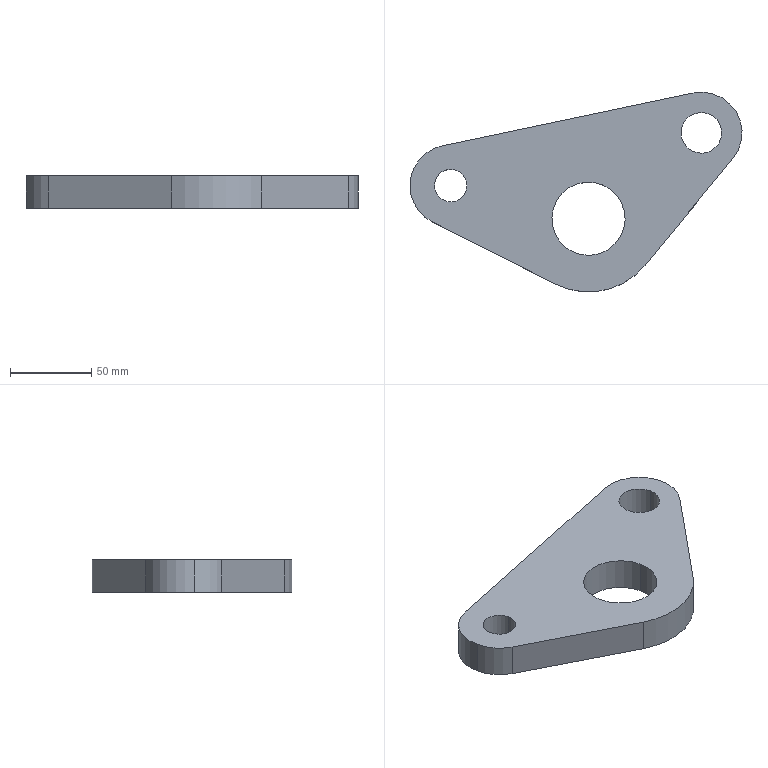Component | SolidWorks | TriangularCrank1-1 | 1 solid | 15 faces | box 204.08 x 122.79 x 20 mm | volume 266584 mm3 | cylinder 10 | plane 5 | commonest cylinder face diameters 50 x3 25 x2 20 x2 45 x2 90 x1 | material N/A
build123d program:
from build123d import *

# Parameters (mm, degrees)
BOSS_EXTRUDE1_DEPTH    = 10
FILLET1_R              = 45
SKETCH2_R              = 22.5
CUT_EXTRUDE1_DEPTH     = 186.55
FILLET2_R              = 25
M20_TAPPED_HOLE1_D     = 20
M20_TAPPED_HOLE1_DEPTH = 47.5
M20_TAPPED_HOLE1_TIP   = 6.009
SKETCH5_R              = 12.5
CUT_EXTRUDE2_DEPTH     = 151.628


with BuildPart() as part:
    # Sketch1 → Boss-Extrude1 (new, symmetric)
    with BuildSketch(Plane(origin=(0, 0, 0), x_dir=(0, 0, -1), z_dir=(1, 0, 0))):
        Polygon((-150, 0), (150, 0), (0, -120), align=None)
    extrude(amount=BOSS_EXTRUDE1_DEPTH, both=True)

    # Fillet1
    fillet1_edges = [part.edges().sort_by_distance(p)[0] for p in [
        (0, -120, 0),
    ]]
    fillet(fillet1_edges, radius=FILLET1_R)

    # Sketch2 → Cut-Extrude1 (cut, through all)
    with BuildSketch(Plane(origin=(10, 0, 0), x_dir=(0, 0, -1), z_dir=(1, 0, 0))):
        with Locations((0, -62.372)):
            Circle(SKETCH2_R)
    extrude(amount=-CUT_EXTRUDE1_DEPTH, mode=Mode.SUBTRACT)

    # Fillet2
    fillet2_edges = [part.edges().sort_by_distance(p)[0] for p in [
        (0, 0, 150),
        (0, 0, -150),
    ]]
    fillet(fillet2_edges, radius=FILLET2_R)

    # M20 Tapped Hole1
    with Locations(Plane(origin=(10, 0, 0), x_dir=(0, 0, -1), z_dir=(1, 0, 0))):
        with Locations((-78.73, -25), (78.73, -25)):
            Hole(M20_TAPPED_HOLE1_D / 2, depth=M20_TAPPED_HOLE1_DEPTH)
            with Locations((0, 0, -(M20_TAPPED_HOLE1_DEPTH + M20_TAPPED_HOLE1_TIP / 2))):  # 118° drill point
                Cone(0, M20_TAPPED_HOLE1_D / 2, M20_TAPPED_HOLE1_TIP, mode=Mode.SUBTRACT)

    # Sketch5 → Cut-Extrude2 (cut, through all)
    with BuildSketch(Plane(origin=(10, 0, 0), x_dir=(0, 0, -1), z_dir=(1, 0, 0))):
        with Locations((78.73, -25)):
            Circle(SKETCH5_R)
    extrude(amount=-CUT_EXTRUDE2_DEPTH, mode=Mode.SUBTRACT)


solid = part.part

# Placed as in the assembly
solid = solid.moved(Location((-12.847, 61.034, 17), (90, -78.113, 90)))
STEP:
#1=COLOUR_RGB('',0.7922,0.8196,0.9333);
#2=FILL_AREA_STYLE_COLOUR('',#1);
#3=FILL_AREA_STYLE('',(#2));
#4=SURFACE_STYLE_FILL_AREA(#3);
#5=SURFACE_SIDE_STYLE('',(#4));
#6=SURFACE_STYLE_USAGE(.BOTH.,#5);
#7=PRESENTATION_STYLE_ASSIGNMENT((#6));
#8=CARTESIAN_POINT('',(2.249,1.977,0.2756));
#9=VERTEX_POINT('',#8);
#10=CARTESIAN_POINT('',(3.212,2.18,0.2756));
#11=VERTEX_POINT('',#10);
#12=CARTESIAN_POINT('',(2.73,2.078,0.2756));
#13=DIRECTION('',(-0.,-0.,1.));
#14=DIRECTION('',(0.9786,0.206,0.));
#15=AXIS2_PLACEMENT_3D('',#12,#13,#14);
#16=CIRCLE('',#15,0.4921);
#17=EDGE_CURVE('',#9,#11,#16,.T.);
#18=ORIENTED_EDGE('',*,*,#17,.F.);
#19=CARTESIAN_POINT('',(2.249,1.977,1.063));
#20=VERTEX_POINT('',#19);
#21=CARTESIAN_POINT('',(2.249,1.977,0.2756));
#22=DIRECTION('',(-0.,-0.,1.));
#23=VECTOR('',#22,39.37);
#24=LINE('',#21,#23);
#25=EDGE_CURVE('',#9,#20,#24,.T.);
#26=ORIENTED_EDGE('',*,*,#25,.T.);
#27=CARTESIAN_POINT('',(3.212,2.18,1.063));
#28=VERTEX_POINT('',#27);
#29=CARTESIAN_POINT('',(2.73,2.078,1.063));
#30=DIRECTION('',(-0.,-0.,1.));
#31=DIRECTION('',(0.9786,0.206,0.));
#32=AXIS2_PLACEMENT_3D('',#29,#30,#31);
#33=CIRCLE('',#32,0.4921);
#34=EDGE_CURVE('',#20,#28,#33,.T.);
#35=ORIENTED_EDGE('',*,*,#34,.T.);
#36=CARTESIAN_POINT('',(3.212,2.18,0.2756));
#37=DIRECTION('',(-0.,-0.,1.));
#38=VECTOR('',#37,39.37);
#39=LINE('',#36,#38);
#40=EDGE_CURVE('',#11,#28,#39,.T.);
#41=ORIENTED_EDGE('',*,*,#40,.F.);
#42=EDGE_LOOP('',(#18,#26,#35,#41));
#43=FACE_OUTER_BOUND('',#42,.T.);
#44=CARTESIAN_POINT('',(2.73,2.078,0.2756));
#45=DIRECTION('',(-0.,-0.,1.));
#46=DIRECTION('',(0.9786,0.206,0.));
#47=AXIS2_PLACEMENT_3D('',#44,#45,#46);
#48=CYLINDRICAL_SURFACE('',#47,0.4921);
#49=ADVANCED_FACE('',(#43),#48,.F.);
#50=CARTESIAN_POINT('',(-2.951,0.8824,0.2756));
#51=VERTEX_POINT('',#50);
#52=CARTESIAN_POINT('',(-3.721,0.7202,0.2756));
#53=VERTEX_POINT('',#52);
#54=CARTESIAN_POINT('',(-3.336,0.8013,0.2756));
#55=DIRECTION('',(0.,0.,-1.));
#56=DIRECTION('',(-0.9786,-0.206,0.));
#57=AXIS2_PLACEMENT_3D('',#54,#55,#56);
#58=CIRCLE('',#57,0.3937);
#59=EDGE_CURVE('',#51,#53,#58,.T.);
#60=ORIENTED_EDGE('',*,*,#59,.T.);
#61=CARTESIAN_POINT('',(-3.721,0.7202,1.063));
#62=VERTEX_POINT('',#61);
#63=CARTESIAN_POINT('',(-3.721,0.7202,1.063));
#64=DIRECTION('',(-0.,-0.,1.));
#65=VECTOR('',#64,39.37);
#66=LINE('',#63,#65);
#67=EDGE_CURVE('',#53,#62,#66,.T.);
#68=ORIENTED_EDGE('',*,*,#67,.T.);
#69=CARTESIAN_POINT('',(-2.951,0.8824,1.063));
#70=VERTEX_POINT('',#69);
#71=CARTESIAN_POINT('',(-3.336,0.8013,1.063));
#72=DIRECTION('',(-0.,-0.,1.));
#73=DIRECTION('',(0.9786,0.206,0.));
#74=AXIS2_PLACEMENT_3D('',#71,#72,#73);
#75=CIRCLE('',#74,0.3937);
#76=EDGE_CURVE('',#62,#70,#75,.T.);
#77=ORIENTED_EDGE('',*,*,#76,.T.);
#78=CARTESIAN_POINT('',(-2.951,0.8824,1.063));
#79=DIRECTION('',(-0.,-0.,1.));
#80=VECTOR('',#79,39.37);
#81=LINE('',#78,#80);
#82=EDGE_CURVE('',#51,#70,#81,.T.);
#83=ORIENTED_EDGE('',*,*,#82,.F.);
#84=EDGE_LOOP('',(#60,#68,#77,#83));
#85=FACE_OUTER_BOUND('',#84,.T.);
#86=CARTESIAN_POINT('',(-3.336,0.8013,1.063));
#87=DIRECTION('',(-0.,-0.,1.));
#88=DIRECTION('',(0.9786,0.206,0.));
#89=AXIS2_PLACEMENT_3D('',#86,#87,#88);
#90=CYLINDRICAL_SURFACE('',#89,0.3937);
#91=ADVANCED_FACE('',(#85),#90,.F.);
#92=CARTESIAN_POINT('',(-4.299,0.5986,1.063));
#93=VERTEX_POINT('',#92);
#94=CARTESIAN_POINT('',(-3.78,-0.07742,1.063));
#95=VERTEX_POINT('',#94);
#96=CARTESIAN_POINT('',(-3.336,0.8013,1.063));
#97=DIRECTION('',(-0.,-0.,1.));
#98=DIRECTION('',(-0.9786,-0.206,0.));
#99=AXIS2_PLACEMENT_3D('',#96,#97,#98);
#100=CIRCLE('',#99,0.9843);
#101=EDGE_CURVE('',#93,#95,#100,.T.);
#102=ORIENTED_EDGE('',*,*,#101,.F.);
#103=CARTESIAN_POINT('',(-4.299,0.5986,0.2756));
#104=VERTEX_POINT('',#103);
#105=CARTESIAN_POINT('',(-4.299,0.5986,1.063));
#106=DIRECTION('',(0.,0.,-1.));
#107=VECTOR('',#106,39.37);
#108=LINE('',#105,#107);
#109=EDGE_CURVE('',#93,#104,#108,.T.);
#110=ORIENTED_EDGE('',*,*,#109,.T.);
#111=CARTESIAN_POINT('',(-3.78,-0.07742,0.2756));
#112=VERTEX_POINT('',#111);
#113=CARTESIAN_POINT('',(-3.336,0.8013,0.2756));
#114=DIRECTION('',(0.,0.,-1.));
#115=DIRECTION('',(-0.9786,-0.206,-0.));
#116=AXIS2_PLACEMENT_3D('',#113,#114,#115);
#117=CIRCLE('',#116,0.9843);
#118=EDGE_CURVE('',#112,#104,#117,.T.);
#119=ORIENTED_EDGE('',*,*,#118,.F.);
#120=CARTESIAN_POINT('',(-3.78,-0.07742,1.063));
#121=DIRECTION('',(0.,0.,-1.));
#122=VECTOR('',#121,39.37);
#123=LINE('',#120,#122);
#124=EDGE_CURVE('',#95,#112,#123,.T.);
#125=ORIENTED_EDGE('',*,*,#124,.F.);
#126=EDGE_LOOP('',(#102,#110,#119,#125));
#127=FACE_OUTER_BOUND('',#126,.T.);
#128=CARTESIAN_POINT('',(-3.336,0.8013,1.063));
#129=DIRECTION('',(0.,0.,-1.));
#130=DIRECTION('',(-0.9786,-0.206,0.));
#131=AXIS2_PLACEMENT_3D('',#128,#129,#130);
#132=CYLINDRICAL_SURFACE('',#131,0.9843);
#133=ADVANCED_FACE('',(#127),#132,.T.);
#134=CARTESIAN_POINT('',(-0.8668,-0.1825,0.2756));
#135=VERTEX_POINT('',#134);
#136=CARTESIAN_POINT('',(0.8668,0.1825,0.2756));
#137=VERTEX_POINT('',#136);
#138=CARTESIAN_POINT('',(-0.,0.,0.2756));
#139=DIRECTION('',(-0.,-0.,1.));
#140=DIRECTION('',(0.9786,0.206,0.));
#141=AXIS2_PLACEMENT_3D('',#138,#139,#140);
#142=CIRCLE('',#141,0.8858);
#143=EDGE_CURVE('',#135,#137,#142,.T.);
#144=ORIENTED_EDGE('',*,*,#143,.F.);
#145=CARTESIAN_POINT('',(-0.8668,-0.1825,1.063));
#146=VERTEX_POINT('',#145);
#147=CARTESIAN_POINT('',(-0.8668,-0.1825,0.2756));
#148=DIRECTION('',(-0.,-0.,1.));
#149=VECTOR('',#148,39.37);
#150=LINE('',#147,#149);
#151=EDGE_CURVE('',#135,#146,#150,.T.);
#152=ORIENTED_EDGE('',*,*,#151,.T.);
#153=CARTESIAN_POINT('',(0.8668,0.1825,1.063));
#154=VERTEX_POINT('',#153);
#155=CARTESIAN_POINT('',(-0.,0.,1.063));
#156=DIRECTION('',(-0.,-0.,1.));
#157=DIRECTION('',(0.9786,0.206,0.));
#158=AXIS2_PLACEMENT_3D('',#155,#156,#157);
#159=CIRCLE('',#158,0.8858);
#160=EDGE_CURVE('',#146,#154,#159,.T.);
#161=ORIENTED_EDGE('',*,*,#160,.T.);
#162=CARTESIAN_POINT('',(0.8668,0.1825,0.2756));
#163=DIRECTION('',(-0.,-0.,1.));
#164=VECTOR('',#163,39.37);
#165=LINE('',#162,#164);
#166=EDGE_CURVE('',#137,#154,#165,.T.);
#167=ORIENTED_EDGE('',*,*,#166,.F.);
#168=EDGE_LOOP('',(#144,#152,#161,#167));
#169=FACE_OUTER_BOUND('',#168,.T.);
#170=CARTESIAN_POINT('',(-0.,0.,0.2756));
#171=DIRECTION('',(-0.,-0.,1.));
#172=DIRECTION('',(0.9786,0.206,0.));
#173=AXIS2_PLACEMENT_3D('',#170,#171,#172);
#174=CYLINDRICAL_SURFACE('',#173,0.8858);
#175=ADVANCED_FACE('',(#169),#174,.F.);
#176=CARTESIAN_POINT('',(1.368,-1.126,0.2756));
#177=VERTEX_POINT('',#176);
#178=CARTESIAN_POINT('',(3.49,1.453,0.2756));
#179=VERTEX_POINT('',#178);
#180=CARTESIAN_POINT('',(5.273,3.619,0.2756));
#181=DIRECTION('',(0.6354,0.7721,0.));
#182=VECTOR('',#181,39.37);
#183=LINE('',#180,#182);
#184=EDGE_CURVE('',#177,#179,#183,.T.);
#185=ORIENTED_EDGE('',*,*,#184,.T.);
#186=CARTESIAN_POINT('',(3.49,1.453,1.063));
#187=VERTEX_POINT('',#186);
#188=CARTESIAN_POINT('',(3.49,1.453,1.063));
#189=DIRECTION('',(-0.,-0.,1.));
#190=VECTOR('',#189,39.37);
#191=LINE('',#188,#190);
#192=EDGE_CURVE('',#179,#187,#191,.T.);
#193=ORIENTED_EDGE('',*,*,#192,.T.);
#194=CARTESIAN_POINT('',(1.368,-1.126,1.063));
#195=VERTEX_POINT('',#194);
#196=CARTESIAN_POINT('',(5.273,3.619,1.063));
#197=DIRECTION('',(0.6354,0.7721,0.));
#198=VECTOR('',#197,39.37);
#199=LINE('',#196,#198);
#200=EDGE_CURVE('',#195,#187,#199,.T.);
#201=ORIENTED_EDGE('',*,*,#200,.F.);
#202=CARTESIAN_POINT('',(1.368,-1.126,1.063));
#203=DIRECTION('',(0.,0.,-1.));
#204=VECTOR('',#203,39.37);
#205=LINE('',#202,#204);
#206=EDGE_CURVE('',#195,#177,#205,.T.);
#207=ORIENTED_EDGE('',*,*,#206,.T.);
#208=EDGE_LOOP('',(#185,#193,#201,#207));
#209=FACE_OUTER_BOUND('',#208,.T.);
#210=CARTESIAN_POINT('',(5.273,3.619,1.063));
#211=DIRECTION('',(-0.7721,0.6354,0.));
#212=DIRECTION('',(-0.6354,-0.7721,-0.));
#213=AXIS2_PLACEMENT_3D('',#210,#211,#212);
#214=PLANE('',#213);
#215=ADVANCED_FACE('',(#209),#214,.F.);
#216=CARTESIAN_POINT('',(2.527,3.041,1.063));
#217=VERTEX_POINT('',#216);
#218=CARTESIAN_POINT('',(-3.539,1.764,1.063));
#219=VERTEX_POINT('',#218);
#220=CARTESIAN_POINT('',(-6.285,1.187,1.063));
#221=DIRECTION('',(-0.9786,-0.206,-0.));
#222=VECTOR('',#221,39.37);
#223=LINE('',#220,#222);
#224=EDGE_CURVE('',#217,#219,#223,.T.);
#225=ORIENTED_EDGE('',*,*,#224,.F.);
#226=CARTESIAN_POINT('',(2.527,3.041,0.2756));
#227=VERTEX_POINT('',#226);
#228=CARTESIAN_POINT('',(2.527,3.041,1.063));
#229=DIRECTION('',(0.,0.,-1.));
#230=VECTOR('',#229,39.37);
#231=LINE('',#228,#230);
#232=EDGE_CURVE('',#217,#227,#231,.T.);
#233=ORIENTED_EDGE('',*,*,#232,.T.);
#234=CARTESIAN_POINT('',(-3.539,1.764,0.2756));
#235=VERTEX_POINT('',#234);
#236=CARTESIAN_POINT('',(-6.285,1.187,0.2756));
#237=DIRECTION('',(-0.9786,-0.206,-0.));
#238=VECTOR('',#237,39.37);
#239=LINE('',#236,#238);
#240=EDGE_CURVE('',#227,#235,#239,.T.);
#241=ORIENTED_EDGE('',*,*,#240,.T.);
#242=CARTESIAN_POINT('',(-3.539,1.764,1.063));
#243=DIRECTION('',(-0.,-0.,1.));
#244=VECTOR('',#243,39.37);
#245=LINE('',#242,#244);
#246=EDGE_CURVE('',#235,#219,#245,.T.);
#247=ORIENTED_EDGE('',*,*,#246,.T.);
#248=EDGE_LOOP('',(#225,#233,#241,#247));
#249=FACE_OUTER_BOUND('',#248,.T.);
#250=CARTESIAN_POINT('',(-6.285,1.187,1.063));
#251=DIRECTION('',(0.206,-0.9786,-0.));
#252=DIRECTION('',(0.9786,0.206,0.));
#253=AXIS2_PLACEMENT_3D('',#250,#251,#252);
#254=PLANE('',#253);
#255=ADVANCED_FACE('',(#249),#254,.F.);
#256=CARTESIAN_POINT('',(-0.7981,-1.582,1.063));
#257=VERTEX_POINT('',#256);
#258=CARTESIAN_POINT('',(0.4673,-2.22,1.063));
#259=DIRECTION('',(0.8928,-0.4505,-0.));
#260=VECTOR('',#259,39.37);
#261=LINE('',#258,#260);
#262=EDGE_CURVE('',#95,#257,#261,.T.);
#263=ORIENTED_EDGE('',*,*,#262,.F.);
#264=ORIENTED_EDGE('',*,*,#124,.T.);
#265=CARTESIAN_POINT('',(-0.7981,-1.582,0.2756));
#266=VERTEX_POINT('',#265);
#267=CARTESIAN_POINT('',(0.4673,-2.22,0.2756));
#268=DIRECTION('',(0.8928,-0.4505,-0.));
#269=VECTOR('',#268,39.37);
#270=LINE('',#267,#269);
#271=EDGE_CURVE('',#112,#266,#270,.T.);
#272=ORIENTED_EDGE('',*,*,#271,.T.);
#273=CARTESIAN_POINT('',(-0.7981,-1.582,1.063));
#274=DIRECTION('',(-0.,-0.,1.));
#275=VECTOR('',#274,39.37);
#276=LINE('',#273,#275);
#277=EDGE_CURVE('',#266,#257,#276,.T.);
#278=ORIENTED_EDGE('',*,*,#277,.T.);
#279=EDGE_LOOP('',(#263,#264,#272,#278));
#280=FACE_OUTER_BOUND('',#279,.T.);
#281=CARTESIAN_POINT('',(0.4673,-2.22,1.063));
#282=DIRECTION('',(0.4505,0.8928,0.));
#283=DIRECTION('',(-0.8928,0.4505,0.));
#284=AXIS2_PLACEMENT_3D('',#281,#282,#283);
#285=PLANE('',#284);
#286=ADVANCED_FACE('',(#280),#285,.F.);
#287=CARTESIAN_POINT('',(2.73,2.078,1.063));
#288=DIRECTION('',(-0.,-0.,1.));
#289=DIRECTION('',(0.9786,0.206,0.));
#290=AXIS2_PLACEMENT_3D('',#287,#288,#289);
#291=CIRCLE('',#290,0.4921);
#292=EDGE_CURVE('',#28,#20,#291,.T.);
#293=ORIENTED_EDGE('',*,*,#292,.F.);
#294=ORIENTED_EDGE('',*,*,#34,.F.);
#295=EDGE_LOOP('',(#293,#294));
#296=FACE_BOUND('',#295,.T.);
#297=CARTESIAN_POINT('',(-3.336,0.8013,1.063));
#298=DIRECTION('',(-0.,-0.,1.));
#299=DIRECTION('',(0.9786,0.206,0.));
#300=AXIS2_PLACEMENT_3D('',#297,#298,#299);
#301=CIRCLE('',#300,0.3937);
#302=EDGE_CURVE('',#70,#62,#301,.T.);
#303=ORIENTED_EDGE('',*,*,#302,.F.);
#304=ORIENTED_EDGE('',*,*,#76,.F.);
#305=EDGE_LOOP('',(#303,#304));
#306=FACE_BOUND('',#305,.T.);
#307=CARTESIAN_POINT('',(-0.,0.,1.063));
#308=DIRECTION('',(-0.,-0.,1.));
#309=DIRECTION('',(0.9786,0.206,0.));
#310=AXIS2_PLACEMENT_3D('',#307,#308,#309);
#311=CIRCLE('',#310,0.8858);
#312=EDGE_CURVE('',#154,#146,#311,.T.);
#313=ORIENTED_EDGE('',*,*,#312,.F.);
#314=ORIENTED_EDGE('',*,*,#160,.F.);
#315=EDGE_LOOP('',(#313,#314));
#316=FACE_BOUND('',#315,.T.);
#317=ORIENTED_EDGE('',*,*,#200,.T.);
#318=CARTESIAN_POINT('',(2.73,2.078,1.063));
#319=DIRECTION('',(-0.,-0.,1.));
#320=DIRECTION('',(-0.9786,-0.206,0.));
#321=AXIS2_PLACEMENT_3D('',#318,#319,#320);
#322=CIRCLE('',#321,0.9843);
#323=EDGE_CURVE('',#187,#217,#322,.T.);
#324=ORIENTED_EDGE('',*,*,#323,.T.);
#325=ORIENTED_EDGE('',*,*,#224,.T.);
#326=CARTESIAN_POINT('',(-3.336,0.8013,1.063));
#327=DIRECTION('',(-0.,-0.,1.));
#328=DIRECTION('',(-0.9786,-0.206,0.));
#329=AXIS2_PLACEMENT_3D('',#326,#327,#328);
#330=CIRCLE('',#329,0.9843);
#331=EDGE_CURVE('',#219,#93,#330,.T.);
#332=ORIENTED_EDGE('',*,*,#331,.T.);
#333=ORIENTED_EDGE('',*,*,#101,.T.);
#334=ORIENTED_EDGE('',*,*,#262,.T.);
#335=CARTESIAN_POINT('',(-0.,0.,1.063));
#336=DIRECTION('',(-0.,-0.,1.));
#337=DIRECTION('',(-0.9786,-0.206,0.));
#338=AXIS2_PLACEMENT_3D('',#335,#336,#337);
#339=CIRCLE('',#338,1.772);
#340=EDGE_CURVE('',#257,#195,#339,.T.);
#341=ORIENTED_EDGE('',*,*,#340,.T.);
#342=EDGE_LOOP('',(#317,#324,#325,#332,#333,#334,#341));
#343=FACE_OUTER_BOUND('',#342,.T.);
#344=CARTESIAN_POINT('',(-0.5058,2.403,1.063));
#345=DIRECTION('',(0.,0.,-1.));
#346=DIRECTION('',(-0.9786,-0.206,-0.));
#347=AXIS2_PLACEMENT_3D('',#344,#345,#346);
#348=PLANE('',#347);
#349=ADVANCED_FACE('',(#296,#306,#316,#343),#348,.F.);
#350=CARTESIAN_POINT('',(2.73,2.078,0.2756));
#351=DIRECTION('',(-0.,-0.,1.));
#352=DIRECTION('',(0.9786,0.206,0.));
#353=AXIS2_PLACEMENT_3D('',#350,#351,#352);
#354=CIRCLE('',#353,0.4921);
#355=EDGE_CURVE('',#11,#9,#354,.T.);
#356=ORIENTED_EDGE('',*,*,#355,.T.);
#357=ORIENTED_EDGE('',*,*,#17,.T.);
#358=EDGE_LOOP('',(#356,#357));
#359=FACE_BOUND('',#358,.T.);
#360=ORIENTED_EDGE('',*,*,#59,.F.);
#361=CARTESIAN_POINT('',(-3.336,0.8013,0.2756));
#362=DIRECTION('',(0.,0.,-1.));
#363=DIRECTION('',(-0.9786,-0.206,0.));
#364=AXIS2_PLACEMENT_3D('',#361,#362,#363);
#365=CIRCLE('',#364,0.3937);
#366=EDGE_CURVE('',#53,#51,#365,.T.);
#367=ORIENTED_EDGE('',*,*,#366,.F.);
#368=EDGE_LOOP('',(#360,#367));
#369=FACE_BOUND('',#368,.T.);
#370=CARTESIAN_POINT('',(-0.,0.,0.2756));
#371=DIRECTION('',(-0.,-0.,1.));
#372=DIRECTION('',(0.9786,0.206,0.));
#373=AXIS2_PLACEMENT_3D('',#370,#371,#372);
#374=CIRCLE('',#373,0.8858);
#375=EDGE_CURVE('',#137,#135,#374,.T.);
#376=ORIENTED_EDGE('',*,*,#375,.T.);
#377=ORIENTED_EDGE('',*,*,#143,.T.);
#378=EDGE_LOOP('',(#376,#377));
#379=FACE_BOUND('',#378,.T.);
#380=ORIENTED_EDGE('',*,*,#240,.F.);
#381=CARTESIAN_POINT('',(2.73,2.078,0.2756));
#382=DIRECTION('',(0.,0.,-1.));
#383=DIRECTION('',(-0.9786,-0.206,-0.));
#384=AXIS2_PLACEMENT_3D('',#381,#382,#383);
#385=CIRCLE('',#384,0.9843);
#386=EDGE_CURVE('',#227,#179,#385,.T.);
#387=ORIENTED_EDGE('',*,*,#386,.T.);
#388=ORIENTED_EDGE('',*,*,#184,.F.);
#389=CARTESIAN_POINT('',(-0.,0.,0.2756));
#390=DIRECTION('',(0.,0.,-1.));
#391=DIRECTION('',(-0.9786,-0.206,-0.));
#392=AXIS2_PLACEMENT_3D('',#389,#390,#391);
#393=CIRCLE('',#392,1.772);
#394=EDGE_CURVE('',#177,#266,#393,.T.);
#395=ORIENTED_EDGE('',*,*,#394,.T.);
#396=ORIENTED_EDGE('',*,*,#271,.F.);
#397=ORIENTED_EDGE('',*,*,#118,.T.);
#398=CARTESIAN_POINT('',(-3.336,0.8013,0.2756));
#399=DIRECTION('',(0.,0.,-1.));
#400=DIRECTION('',(-0.9786,-0.206,-0.));
#401=AXIS2_PLACEMENT_3D('',#398,#399,#400);
#402=CIRCLE('',#401,0.9843);
#403=EDGE_CURVE('',#104,#235,#402,.T.);
#404=ORIENTED_EDGE('',*,*,#403,.T.);
#405=EDGE_LOOP('',(#380,#387,#388,#395,#396,#397,#404));
#406=FACE_OUTER_BOUND('',#405,.T.);
#407=CARTESIAN_POINT('',(-0.5058,2.403,0.2756));
#408=DIRECTION('',(0.,0.,-1.));
#409=DIRECTION('',(-0.9786,-0.206,-0.));
#410=AXIS2_PLACEMENT_3D('',#407,#408,#409);
#411=PLANE('',#410);
#412=ADVANCED_FACE('',(#359,#369,#379,#406),#411,.T.);
#413=ORIENTED_EDGE('',*,*,#340,.F.);
#414=ORIENTED_EDGE('',*,*,#277,.F.);
#415=ORIENTED_EDGE('',*,*,#394,.F.);
#416=ORIENTED_EDGE('',*,*,#206,.F.);
#417=EDGE_LOOP('',(#413,#414,#415,#416));
#418=FACE_OUTER_BOUND('',#417,.T.);
#419=CARTESIAN_POINT('',(-0.,0.,1.063));
#420=DIRECTION('',(0.,0.,-1.));
#421=DIRECTION('',(-0.9786,-0.206,0.));
#422=AXIS2_PLACEMENT_3D('',#419,#420,#421);
#423=CYLINDRICAL_SURFACE('',#422,1.772);
#424=ADVANCED_FACE('',(#418),#423,.T.);
#425=ORIENTED_EDGE('',*,*,#151,.F.);
#426=ORIENTED_EDGE('',*,*,#375,.F.);
#427=ORIENTED_EDGE('',*,*,#166,.T.);
#428=ORIENTED_EDGE('',*,*,#312,.T.);
#429=EDGE_LOOP('',(#425,#426,#427,#428));
#430=FACE_OUTER_BOUND('',#429,.T.);
#431=CARTESIAN_POINT('',(-0.,0.,0.2756));
#432=DIRECTION('',(-0.,-0.,1.));
#433=DIRECTION('',(0.9786,0.206,0.));
#434=AXIS2_PLACEMENT_3D('',#431,#432,#433);
#435=CYLINDRICAL_SURFACE('',#434,0.8858);
#436=ADVANCED_FACE('',(#430),#435,.F.);
#437=ORIENTED_EDGE('',*,*,#323,.F.);
#438=ORIENTED_EDGE('',*,*,#192,.F.);
#439=ORIENTED_EDGE('',*,*,#386,.F.);
#440=ORIENTED_EDGE('',*,*,#232,.F.);
#441=EDGE_LOOP('',(#437,#438,#439,#440));
#442=FACE_OUTER_BOUND('',#441,.T.);
#443=CARTESIAN_POINT('',(2.73,2.078,1.063));
#444=DIRECTION('',(0.,0.,-1.));
#445=DIRECTION('',(-0.9786,-0.206,0.));
#446=AXIS2_PLACEMENT_3D('',#443,#444,#445);
#447=CYLINDRICAL_SURFACE('',#446,0.9843);
#448=ADVANCED_FACE('',(#442),#447,.T.);
#449=ORIENTED_EDGE('',*,*,#109,.F.);
#450=ORIENTED_EDGE('',*,*,#331,.F.);
#451=ORIENTED_EDGE('',*,*,#246,.F.);
#452=ORIENTED_EDGE('',*,*,#403,.F.);
#453=EDGE_LOOP('',(#449,#450,#451,#452));
#454=FACE_OUTER_BOUND('',#453,.T.);
#455=CARTESIAN_POINT('',(-3.336,0.8013,1.063));
#456=DIRECTION('',(0.,0.,-1.));
#457=DIRECTION('',(-0.9786,-0.206,0.));
#458=AXIS2_PLACEMENT_3D('',#455,#456,#457);
#459=CYLINDRICAL_SURFACE('',#458,0.9843);
#460=ADVANCED_FACE('',(#454),#459,.T.);
#461=ORIENTED_EDGE('',*,*,#67,.F.);
#462=ORIENTED_EDGE('',*,*,#366,.T.);
#463=ORIENTED_EDGE('',*,*,#82,.T.);
#464=ORIENTED_EDGE('',*,*,#302,.T.);
#465=EDGE_LOOP('',(#461,#462,#463,#464));
#466=FACE_OUTER_BOUND('',#465,.T.);
#467=CARTESIAN_POINT('',(-3.336,0.8013,1.063));
#468=DIRECTION('',(-0.,-0.,1.));
#469=DIRECTION('',(0.9786,0.206,0.));
#470=AXIS2_PLACEMENT_3D('',#467,#468,#469);
#471=CYLINDRICAL_SURFACE('',#470,0.3937);
#472=ADVANCED_FACE('',(#466),#471,.F.);
#473=ORIENTED_EDGE('',*,*,#25,.F.);
#474=ORIENTED_EDGE('',*,*,#355,.F.);
#475=ORIENTED_EDGE('',*,*,#40,.T.);
#476=ORIENTED_EDGE('',*,*,#292,.T.);
#477=EDGE_LOOP('',(#473,#474,#475,#476));
#478=FACE_OUTER_BOUND('',#477,.T.);
#479=CARTESIAN_POINT('',(2.73,2.078,0.2756));
#480=DIRECTION('',(-0.,-0.,1.));
#481=DIRECTION('',(0.9786,0.206,0.));
#482=AXIS2_PLACEMENT_3D('',#479,#480,#481);
#483=CYLINDRICAL_SURFACE('',#482,0.4921);
#484=ADVANCED_FACE('',(#478),#483,.F.);
#485=CLOSED_SHELL('',(#49,#91,#133,#175,#215,#255,#286,#349,#412,#424,#436,#448,#460,#472,#484));
#486=MANIFOLD_SOLID_BREP('',#485);
#487=STYLED_ITEM('',(#7),#486);
#488=(LENGTH_UNIT()NAMED_UNIT(*)SI_UNIT($,.METRE.));
#489=LENGTH_MEASURE_WITH_UNIT(LENGTH_MEASURE(0.0254),#488);
#490=DIMENSIONAL_EXPONENTS(1.,0.,0.,0.,0.,0.,0.);
#491=(CONVERSION_BASED_UNIT('',#489)LENGTH_UNIT()NAMED_UNIT(#490));
#492=UNCERTAINTY_MEASURE_WITH_UNIT(LENGTH_MEASURE(0.00001),#491,'','');
#493=(NAMED_UNIT(*)PLANE_ANGLE_UNIT()SI_UNIT($,.RADIAN.));
#494=(NAMED_UNIT(*)SI_UNIT($,.STERADIAN.)SOLID_ANGLE_UNIT());
#495=(GEOMETRIC_REPRESENTATION_CONTEXT(3)GLOBAL_UNCERTAINTY_ASSIGNED_CONTEXT((#492))GLOBAL_UNIT_ASSIGNED_CONTEXT((#491,#493,#494))REPRESENTATION_CONTEXT('',''));
#496=MECHANICAL_DESIGN_GEOMETRIC_PRESENTATION_REPRESENTATION('',(#487),#495);
#497=CARTESIAN_POINT('',(0.,0.,0.));
#498=DIRECTION('',(0.,0.,1.));
#499=DIRECTION('',(1.,0.,0.));
#500=AXIS2_PLACEMENT_3D('',#497,#498,#499);
#501=(LENGTH_UNIT()NAMED_UNIT(*)SI_UNIT($,.METRE.));
#502=LENGTH_MEASURE_WITH_UNIT(LENGTH_MEASURE(0.0254),#501);
#503=DIMENSIONAL_EXPONENTS(1.,0.,0.,0.,0.,0.,0.);
#504=(CONVERSION_BASED_UNIT('',#502)LENGTH_UNIT()NAMED_UNIT(#503));
#505=UNCERTAINTY_MEASURE_WITH_UNIT(LENGTH_MEASURE(0.00001),#504,'','');
#506=(NAMED_UNIT(*)PLANE_ANGLE_UNIT()SI_UNIT($,.RADIAN.));
#507=(NAMED_UNIT(*)SI_UNIT($,.STERADIAN.)SOLID_ANGLE_UNIT());
#508=(GEOMETRIC_REPRESENTATION_CONTEXT(3)GLOBAL_UNCERTAINTY_ASSIGNED_CONTEXT((#505))GLOBAL_UNIT_ASSIGNED_CONTEXT((#504,#506,#507))REPRESENTATION_CONTEXT('',''));
#509=ADVANCED_BREP_SHAPE_REPRESENTATION('',(#486,#500),#508);
#510=PRESENTATION_LAYER_ASSIGNMENT('','',(#487));